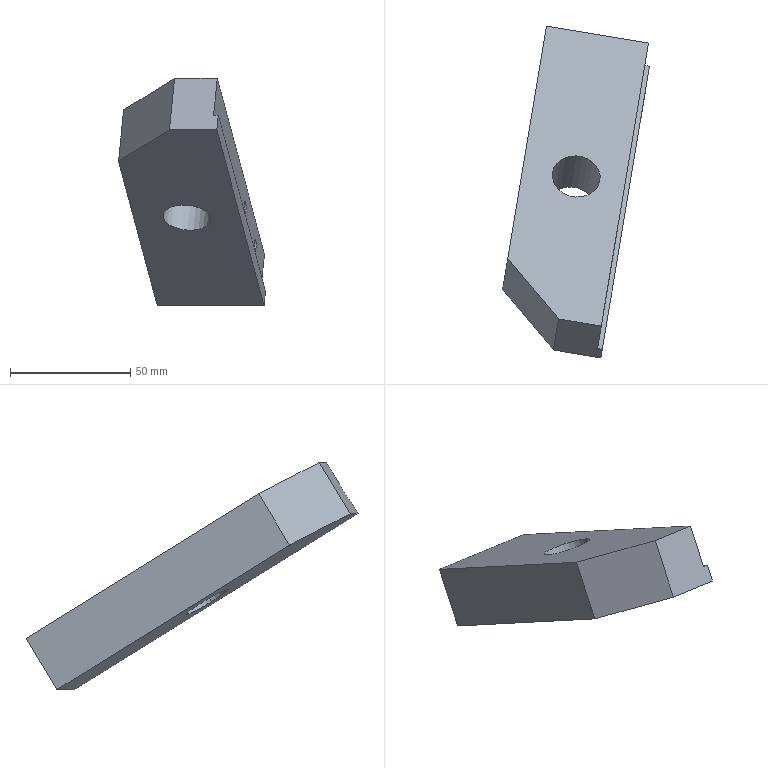Component | SolidWorks | 14AC-24-1-006-1 | 1 solid | 35 faces | box 61.1 x 138.05 x 94.42 mm | volume 135396 mm3 | cylinder 14 | cone 12 | plane 9 | commonest cylinder face diameters 4.2 x8 5 x4 20 x2
build123d program:
from build123d import *

# Parameters (mm, degrees)
SKETCH1_W             = 45
SKETCH1_H             = 140
BOSS_EXTRUDE1_DEPTH   = 25
CUT_EXTRUDE2_DEPTH    = 2
CHAMFER2_SIZE         = 25
M6_TAPPED_HOLE1_D     = 5
M6_TAPPED_HOLE1_DEPTH = 17
M6_TAPPED_HOLE1_TIP   = 1.502
M5_TAPPED_HOLE2_D     = 4.2
M5_TAPPED_HOLE2_DEPTH = 12.4
M5_TAPPED_HOLE2_TIP   = 1.262
SKETCH8_R             = 10
CUT_EXTRUDE3_DEPTH    = 78.661


with BuildPart() as part:
    # Sketch1 → Boss-Extrude1 (new body)
    with BuildSketch(Plane.XY):
        Rectangle(SKETCH1_W, SKETCH1_H)
    extrude(amount=BOSS_EXTRUDE1_DEPTH)

    # Sketch4 → Cut-Extrude2 (cut)
    with BuildSketch(Plane(origin=(22.5, 0, 0), x_dir=(0, 0, -1), z_dir=(1, 0, 0))):
        with BuildLine():
            Line((-18, 70), (0, 70))
            Line((0, 70), (0, -78.5))
            ThreePointArc((0, -78.5), (1.061, -81.061), (-1.5, -80))
            Line((-1.5, -80), (-16.5, -80))
            ThreePointArc((-16.5, -80), (-19.061, -81.061), (-18, -78.5))
            Line((-18, -78.5), (-18, 70))
        make_face()
    extrude(amount=-CUT_EXTRUDE2_DEPTH, mode=Mode.SUBTRACT)

    # Chamfer2
    chamfer2_edges = [part.edges().sort_by_distance(p)[0] for p in [
        (-22.5, 70, 12.5),
    ]]
    chamfer(chamfer2_edges, length=CHAMFER2_SIZE)

    # M6 Tapped Hole1
    with Locations(Plane(origin=(20.5, -48, 9), x_dir=(0, 1, 0), z_dir=(1, 0, 0))):
        with Locations((0, 0), (30, 0)):
            Hole(M6_TAPPED_HOLE1_D / 2, depth=M6_TAPPED_HOLE1_DEPTH)
            with Locations((0, 0, -(M6_TAPPED_HOLE1_DEPTH + M6_TAPPED_HOLE1_TIP / 2))):  # 118° drill point
                Cone(0, M6_TAPPED_HOLE1_D / 2, M6_TAPPED_HOLE1_TIP, mode=Mode.SUBTRACT)

    # M5 Tapped Hole2
    with Locations(Plane(origin=(0, -70, 0), x_dir=(-1, 0, 0), z_dir=(0, -1, 0))):
        with Locations((-12, -4.5), (14, -4.5), (14, -20.5), (-12, -20.5)):
            Hole(M5_TAPPED_HOLE2_D / 2, depth=M5_TAPPED_HOLE2_DEPTH)
            with Locations((0, 0, -(M5_TAPPED_HOLE2_DEPTH + M5_TAPPED_HOLE2_TIP / 2))):  # 118° drill point
                Cone(0, M5_TAPPED_HOLE2_D / 2, M5_TAPPED_HOLE2_TIP, mode=Mode.SUBTRACT)

    # Sketch8 → Cut-Extrude3 (cut, through all)
    with BuildSketch(Plane.XY.offset(25)):
        Circle(SKETCH8_R)
    extrude(amount=-CUT_EXTRUDE3_DEPTH, mode=Mode.SUBTRACT)


solid = part.part

# Placed as in the assembly
solid = solid.moved(Location((401.932, -204.897, -116.607), (148.871, -4.92, 8.082)))
STEP:
#1=COLOUR_RGB('',0.7922,0.8196,0.9333);
#2=FILL_AREA_STYLE_COLOUR('',#1);
#3=FILL_AREA_STYLE('',(#2));
#4=SURFACE_STYLE_FILL_AREA(#3);
#5=SURFACE_SIDE_STYLE('',(#4));
#6=SURFACE_STYLE_USAGE(.BOTH.,#5);
#7=PRESENTATION_STYLE_ASSIGNMENT((#6));
#8=CARTESIAN_POINT('',(15.436,-8.002,-4.591));
#9=VERTEX_POINT('',#8);
#10=CARTESIAN_POINT('',(16.212,-8.131,-4.591));
#11=VERTEX_POINT('',#10);
#12=CARTESIAN_POINT('',(15.824,-8.067,-4.591));
#13=DIRECTION('',(-0.08576,-0.5151,-0.8529));
#14=DIRECTION('',(0.9864,-0.1642,-0.));
#15=AXIS2_PLACEMENT_3D('',#12,#13,#14);
#16=CIRCLE('',#15,0.3937);
#17=EDGE_CURVE('',#9,#11,#16,.T.);
#18=ORIENTED_EDGE('',*,*,#17,.F.);
#19=CARTESIAN_POINT('',(15.351,-8.509,-5.43));
#20=VERTEX_POINT('',#19);
#21=CARTESIAN_POINT('',(15.436,-8.002,-4.591));
#22=DIRECTION('',(-0.08576,-0.5151,-0.8529));
#23=VECTOR('',#22,39.37);
#24=LINE('',#21,#23);
#25=EDGE_CURVE('',#9,#20,#24,.T.);
#26=ORIENTED_EDGE('',*,*,#25,.T.);
#27=CARTESIAN_POINT('',(16.128,-8.638,-5.43));
#28=VERTEX_POINT('',#27);
#29=CARTESIAN_POINT('',(15.74,-8.574,-5.43));
#30=DIRECTION('',(-0.08576,-0.5151,-0.8529));
#31=DIRECTION('',(0.9864,-0.1642,0.));
#32=AXIS2_PLACEMENT_3D('',#29,#30,#31);
#33=CIRCLE('',#32,0.3937);
#34=EDGE_CURVE('',#20,#28,#33,.T.);
#35=ORIENTED_EDGE('',*,*,#34,.T.);
#36=CARTESIAN_POINT('',(16.212,-8.131,-4.591));
#37=DIRECTION('',(-0.08576,-0.5151,-0.8529));
#38=VECTOR('',#37,39.37);
#39=LINE('',#36,#38);
#40=EDGE_CURVE('',#11,#28,#39,.T.);
#41=ORIENTED_EDGE('',*,*,#40,.F.);
#42=EDGE_LOOP('',(#18,#26,#35,#41));
#43=FACE_OUTER_BOUND('',#42,.T.);
#44=CARTESIAN_POINT('',(15.824,-8.067,-4.591));
#45=DIRECTION('',(-0.08576,-0.5151,-0.8529));
#46=DIRECTION('',(0.9864,-0.1642,-0.));
#47=AXIS2_PLACEMENT_3D('',#44,#45,#46);
#48=CYLINDRICAL_SURFACE('',#47,0.3937);
#49=ADVANCED_FACE('',(#43),#48,.F.);
#50=CARTESIAN_POINT('',(16.586,-6.37,-5.997));
#51=VERTEX_POINT('',#50);
#52=CARTESIAN_POINT('',(16.6,-6.285,-5.855));
#53=VERTEX_POINT('',#52);
#54=CARTESIAN_POINT('',(16.593,-6.328,-5.926));
#55=DIRECTION('',(0.1401,0.8413,-0.5222));
#56=DIRECTION('',(0.08576,0.5151,0.8529));
#57=AXIS2_PLACEMENT_3D('',#54,#55,#56);
#58=CIRCLE('',#57,0.08268);
#59=EDGE_CURVE('',#51,#53,#58,.T.);
#60=ORIENTED_EDGE('',*,*,#59,.F.);
#61=CARTESIAN_POINT('',(16.654,-5.96,-6.251));
#62=VERTEX_POINT('',#61);
#63=CARTESIAN_POINT('',(16.654,-5.96,-6.251));
#64=DIRECTION('',(0.1401,0.8413,-0.5222));
#65=VECTOR('',#64,39.37);
#66=LINE('',#63,#65);
#67=EDGE_CURVE('',#51,#62,#66,.T.);
#68=ORIENTED_EDGE('',*,*,#67,.T.);
#69=CARTESIAN_POINT('',(16.668,-5.875,-6.11));
#70=VERTEX_POINT('',#69);
#71=CARTESIAN_POINT('',(16.661,-5.917,-6.181));
#72=DIRECTION('',(0.1401,0.8413,-0.5222));
#73=DIRECTION('',(0.08576,0.5151,0.8529));
#74=AXIS2_PLACEMENT_3D('',#71,#72,#73);
#75=CIRCLE('',#74,0.08268);
#76=EDGE_CURVE('',#62,#70,#75,.T.);
#77=ORIENTED_EDGE('',*,*,#76,.T.);
#78=CARTESIAN_POINT('',(16.668,-5.875,-6.11));
#79=DIRECTION('',(0.1401,0.8413,-0.5222));
#80=VECTOR('',#79,39.37);
#81=LINE('',#78,#80);
#82=EDGE_CURVE('',#53,#70,#81,.T.);
#83=ORIENTED_EDGE('',*,*,#82,.F.);
#84=EDGE_LOOP('',(#60,#68,#77,#83));
#85=FACE_OUTER_BOUND('',#84,.T.);
#86=CARTESIAN_POINT('',(16.661,-5.917,-6.181));
#87=DIRECTION('',(0.1401,0.8413,-0.5222));
#88=DIRECTION('',(0.08576,0.5151,0.8529));
#89=AXIS2_PLACEMENT_3D('',#86,#87,#88);
#90=CYLINDRICAL_SURFACE('',#89,0.08268);
#91=ADVANCED_FACE('',(#85),#90,.F.);
#92=CARTESIAN_POINT('',(16.586,-6.37,-5.9));
#93=VERTEX_POINT('',#92);
#94=CARTESIAN_POINT('',(16.6,-6.285,-5.855));
#95=DIRECTION('',(0.1457,0.8748,0.4621));
#96=VECTOR('',#95,39.37);
#97=LINE('',#94,#96);
#98=EDGE_CURVE('',#93,#53,#97,.T.);
#99=ORIENTED_EDGE('',*,*,#98,.F.);
#100=CARTESIAN_POINT('',(16.586,-6.37,-5.997));
#101=DIRECTION('',(-0.001367,-0.008211,-1.));
#102=VECTOR('',#101,39.37);
#103=LINE('',#100,#102);
#104=EDGE_CURVE('',#93,#51,#103,.T.);
#105=ORIENTED_EDGE('',*,*,#104,.T.);
#106=ORIENTED_EDGE('',*,*,#59,.T.);
#107=EDGE_LOOP('',(#99,#105,#106));
#108=FACE_OUTER_BOUND('',#107,.T.);
#109=CARTESIAN_POINT('',(16.593,-6.328,-5.926));
#110=DIRECTION('',(0.1401,0.8413,-0.5222));
#111=DIRECTION('',(0.08576,0.5151,0.8529));
#112=AXIS2_PLACEMENT_3D('',#109,#110,#111);
#113=CONICAL_SURFACE('',#112,0.08268,1.03);
#114=ADVANCED_FACE('',(#108),#113,.F.);
#115=CARTESIAN_POINT('',(15.576,-6.202,-5.997));
#116=VERTEX_POINT('',#115);
#117=CARTESIAN_POINT('',(15.59,-6.117,-5.855));
#118=VERTEX_POINT('',#117);
#119=CARTESIAN_POINT('',(15.583,-6.16,-5.926));
#120=DIRECTION('',(0.1401,0.8413,-0.5222));
#121=DIRECTION('',(0.08576,0.5151,0.8529));
#122=AXIS2_PLACEMENT_3D('',#119,#120,#121);
#123=CIRCLE('',#122,0.08268);
#124=EDGE_CURVE('',#116,#118,#123,.T.);
#125=ORIENTED_EDGE('',*,*,#124,.F.);
#126=CARTESIAN_POINT('',(15.644,-5.792,-6.251));
#127=VERTEX_POINT('',#126);
#128=CARTESIAN_POINT('',(15.644,-5.792,-6.251));
#129=DIRECTION('',(0.1401,0.8413,-0.5222));
#130=VECTOR('',#129,39.37);
#131=LINE('',#128,#130);
#132=EDGE_CURVE('',#116,#127,#131,.T.);
#133=ORIENTED_EDGE('',*,*,#132,.T.);
#134=CARTESIAN_POINT('',(15.658,-5.707,-6.11));
#135=VERTEX_POINT('',#134);
#136=CARTESIAN_POINT('',(15.651,-5.749,-6.181));
#137=DIRECTION('',(0.1401,0.8413,-0.5222));
#138=DIRECTION('',(0.08576,0.5151,0.8529));
#139=AXIS2_PLACEMENT_3D('',#136,#137,#138);
#140=CIRCLE('',#139,0.08268);
#141=EDGE_CURVE('',#127,#135,#140,.T.);
#142=ORIENTED_EDGE('',*,*,#141,.T.);
#143=CARTESIAN_POINT('',(15.658,-5.707,-6.11));
#144=DIRECTION('',(0.1401,0.8413,-0.5222));
#145=VECTOR('',#144,39.37);
#146=LINE('',#143,#145);
#147=EDGE_CURVE('',#118,#135,#146,.T.);
#148=ORIENTED_EDGE('',*,*,#147,.F.);
#149=EDGE_LOOP('',(#125,#133,#142,#148));
#150=FACE_OUTER_BOUND('',#149,.T.);
#151=CARTESIAN_POINT('',(15.651,-5.749,-6.181));
#152=DIRECTION('',(0.1401,0.8413,-0.5222));
#153=DIRECTION('',(0.08576,0.5151,0.8529));
#154=AXIS2_PLACEMENT_3D('',#151,#152,#153);
#155=CYLINDRICAL_SURFACE('',#154,0.08268);
#156=ADVANCED_FACE('',(#150),#155,.F.);
#157=CARTESIAN_POINT('',(15.576,-6.202,-5.9));
#158=VERTEX_POINT('',#157);
#159=CARTESIAN_POINT('',(15.59,-6.117,-5.855));
#160=DIRECTION('',(0.1457,0.8748,0.4621));
#161=VECTOR('',#160,39.37);
#162=LINE('',#159,#161);
#163=EDGE_CURVE('',#158,#118,#162,.T.);
#164=ORIENTED_EDGE('',*,*,#163,.F.);
#165=CARTESIAN_POINT('',(15.576,-6.202,-5.997));
#166=DIRECTION('',(-0.001367,-0.008211,-1.));
#167=VECTOR('',#166,39.37);
#168=LINE('',#165,#167);
#169=EDGE_CURVE('',#158,#116,#168,.T.);
#170=ORIENTED_EDGE('',*,*,#169,.T.);
#171=ORIENTED_EDGE('',*,*,#124,.T.);
#172=EDGE_LOOP('',(#164,#170,#171));
#173=FACE_OUTER_BOUND('',#172,.T.);
#174=CARTESIAN_POINT('',(15.583,-6.16,-5.926));
#175=DIRECTION('',(0.1401,0.8413,-0.5222));
#176=DIRECTION('',(0.08576,0.5151,0.8529));
#177=AXIS2_PLACEMENT_3D('',#174,#175,#176);
#178=CONICAL_SURFACE('',#177,0.08268,1.03);
#179=ADVANCED_FACE('',(#173),#178,.F.);
#180=CARTESIAN_POINT('',(15.522,-6.527,-6.534));
#181=VERTEX_POINT('',#180);
#182=CARTESIAN_POINT('',(15.536,-6.442,-6.393));
#183=VERTEX_POINT('',#182);
#184=CARTESIAN_POINT('',(15.529,-6.484,-6.463));
#185=DIRECTION('',(0.1401,0.8413,-0.5222));
#186=DIRECTION('',(0.08576,0.5151,0.8529));
#187=AXIS2_PLACEMENT_3D('',#184,#185,#186);
#188=CIRCLE('',#187,0.08268);
#189=EDGE_CURVE('',#181,#183,#188,.T.);
#190=ORIENTED_EDGE('',*,*,#189,.F.);
#191=CARTESIAN_POINT('',(15.59,-6.116,-6.789));
#192=VERTEX_POINT('',#191);
#193=CARTESIAN_POINT('',(15.59,-6.116,-6.789));
#194=DIRECTION('',(0.1401,0.8413,-0.5222));
#195=VECTOR('',#194,39.37);
#196=LINE('',#193,#195);
#197=EDGE_CURVE('',#181,#192,#196,.T.);
#198=ORIENTED_EDGE('',*,*,#197,.T.);
#199=CARTESIAN_POINT('',(15.604,-6.031,-6.648));
#200=VERTEX_POINT('',#199);
#201=CARTESIAN_POINT('',(15.597,-6.074,-6.718));
#202=DIRECTION('',(0.1401,0.8413,-0.5222));
#203=DIRECTION('',(0.08576,0.5151,0.8529));
#204=AXIS2_PLACEMENT_3D('',#201,#202,#203);
#205=CIRCLE('',#204,0.08268);
#206=EDGE_CURVE('',#192,#200,#205,.T.);
#207=ORIENTED_EDGE('',*,*,#206,.T.);
#208=CARTESIAN_POINT('',(15.604,-6.031,-6.648));
#209=DIRECTION('',(0.1401,0.8413,-0.5222));
#210=VECTOR('',#209,39.37);
#211=LINE('',#208,#210);
#212=EDGE_CURVE('',#183,#200,#211,.T.);
#213=ORIENTED_EDGE('',*,*,#212,.F.);
#214=EDGE_LOOP('',(#190,#198,#207,#213));
#215=FACE_OUTER_BOUND('',#214,.T.);
#216=CARTESIAN_POINT('',(15.597,-6.074,-6.718));
#217=DIRECTION('',(0.1401,0.8413,-0.5222));
#218=DIRECTION('',(0.08576,0.5151,0.8529));
#219=AXIS2_PLACEMENT_3D('',#216,#217,#218);
#220=CYLINDRICAL_SURFACE('',#219,0.08268);
#221=ADVANCED_FACE('',(#215),#220,.F.);
#222=CARTESIAN_POINT('',(15.522,-6.526,-6.437));
#223=VERTEX_POINT('',#222);
#224=CARTESIAN_POINT('',(15.536,-6.442,-6.393));
#225=DIRECTION('',(0.1457,0.8748,0.4621));
#226=VECTOR('',#225,39.37);
#227=LINE('',#224,#226);
#228=EDGE_CURVE('',#223,#183,#227,.T.);
#229=ORIENTED_EDGE('',*,*,#228,.F.);
#230=CARTESIAN_POINT('',(15.522,-6.527,-6.534));
#231=DIRECTION('',(-0.001367,-0.008211,-1.));
#232=VECTOR('',#231,39.37);
#233=LINE('',#230,#232);
#234=EDGE_CURVE('',#223,#181,#233,.T.);
#235=ORIENTED_EDGE('',*,*,#234,.T.);
#236=ORIENTED_EDGE('',*,*,#189,.T.);
#237=EDGE_LOOP('',(#229,#235,#236));
#238=FACE_OUTER_BOUND('',#237,.T.);
#239=CARTESIAN_POINT('',(15.529,-6.484,-6.463));
#240=DIRECTION('',(0.1401,0.8413,-0.5222));
#241=DIRECTION('',(0.08576,0.5151,0.8529));
#242=AXIS2_PLACEMENT_3D('',#239,#240,#241);
#243=CONICAL_SURFACE('',#242,0.08268,1.03);
#244=ADVANCED_FACE('',(#238),#243,.F.);
#245=CARTESIAN_POINT('',(16.531,-6.695,-6.534));
#246=VERTEX_POINT('',#245);
#247=CARTESIAN_POINT('',(16.546,-6.61,-6.393));
#248=VERTEX_POINT('',#247);
#249=CARTESIAN_POINT('',(16.539,-6.652,-6.463));
#250=DIRECTION('',(0.1401,0.8413,-0.5222));
#251=DIRECTION('',(0.08576,0.5151,0.8529));
#252=AXIS2_PLACEMENT_3D('',#249,#250,#251);
#253=CIRCLE('',#252,0.08268);
#254=EDGE_CURVE('',#246,#248,#253,.T.);
#255=ORIENTED_EDGE('',*,*,#254,.F.);
#256=CARTESIAN_POINT('',(16.6,-6.284,-6.789));
#257=VERTEX_POINT('',#256);
#258=CARTESIAN_POINT('',(16.6,-6.284,-6.789));
#259=DIRECTION('',(0.1401,0.8413,-0.5222));
#260=VECTOR('',#259,39.37);
#261=LINE('',#258,#260);
#262=EDGE_CURVE('',#246,#257,#261,.T.);
#263=ORIENTED_EDGE('',*,*,#262,.T.);
#264=CARTESIAN_POINT('',(16.614,-6.199,-6.648));
#265=VERTEX_POINT('',#264);
#266=CARTESIAN_POINT('',(16.607,-6.242,-6.718));
#267=DIRECTION('',(0.1401,0.8413,-0.5222));
#268=DIRECTION('',(0.08576,0.5151,0.8529));
#269=AXIS2_PLACEMENT_3D('',#266,#267,#268);
#270=CIRCLE('',#269,0.08268);
#271=EDGE_CURVE('',#257,#265,#270,.T.);
#272=ORIENTED_EDGE('',*,*,#271,.T.);
#273=CARTESIAN_POINT('',(16.614,-6.199,-6.648));
#274=DIRECTION('',(0.1401,0.8413,-0.5222));
#275=VECTOR('',#274,39.37);
#276=LINE('',#273,#275);
#277=EDGE_CURVE('',#248,#265,#276,.T.);
#278=ORIENTED_EDGE('',*,*,#277,.F.);
#279=EDGE_LOOP('',(#255,#263,#272,#278));
#280=FACE_OUTER_BOUND('',#279,.T.);
#281=CARTESIAN_POINT('',(16.607,-6.242,-6.718));
#282=DIRECTION('',(0.1401,0.8413,-0.5222));
#283=DIRECTION('',(0.08576,0.5151,0.8529));
#284=AXIS2_PLACEMENT_3D('',#281,#282,#283);
#285=CYLINDRICAL_SURFACE('',#284,0.08268);
#286=ADVANCED_FACE('',(#280),#285,.F.);
#287=CARTESIAN_POINT('',(16.532,-6.694,-6.437));
#288=VERTEX_POINT('',#287);
#289=CARTESIAN_POINT('',(16.546,-6.61,-6.393));
#290=DIRECTION('',(0.1457,0.8748,0.4621));
#291=VECTOR('',#290,39.37);
#292=LINE('',#289,#291);
#293=EDGE_CURVE('',#288,#248,#292,.T.);
#294=ORIENTED_EDGE('',*,*,#293,.F.);
#295=CARTESIAN_POINT('',(16.531,-6.695,-6.534));
#296=DIRECTION('',(-0.001367,-0.008211,-1.));
#297=VECTOR('',#296,39.37);
#298=LINE('',#295,#297);
#299=EDGE_CURVE('',#288,#246,#298,.T.);
#300=ORIENTED_EDGE('',*,*,#299,.T.);
#301=ORIENTED_EDGE('',*,*,#254,.T.);
#302=EDGE_LOOP('',(#294,#300,#301));
#303=FACE_OUTER_BOUND('',#302,.T.);
#304=CARTESIAN_POINT('',(16.539,-6.652,-6.463));
#305=DIRECTION('',(0.1401,0.8413,-0.5222));
#306=DIRECTION('',(0.08576,0.5151,0.8529));
#307=AXIS2_PLACEMENT_3D('',#304,#305,#306);
#308=CONICAL_SURFACE('',#307,0.08268,1.03);
#309=ADVANCED_FACE('',(#303),#308,.F.);
#310=CARTESIAN_POINT('',(16.186,-6.733,-5.964));
#311=VERTEX_POINT('',#310);
#312=CARTESIAN_POINT('',(16.203,-6.631,-5.796));
#313=VERTEX_POINT('',#312);
#314=CARTESIAN_POINT('',(16.194,-6.682,-5.88));
#315=DIRECTION('',(0.9864,-0.1642,-0.));
#316=DIRECTION('',(0.08576,0.5151,0.8529));
#317=AXIS2_PLACEMENT_3D('',#314,#315,#316);
#318=CIRCLE('',#317,0.09843);
#319=EDGE_CURVE('',#311,#313,#318,.T.);
#320=ORIENTED_EDGE('',*,*,#319,.F.);
#321=CARTESIAN_POINT('',(16.846,-6.843,-5.964));
#322=VERTEX_POINT('',#321);
#323=CARTESIAN_POINT('',(16.846,-6.843,-5.964));
#324=DIRECTION('',(0.9864,-0.1642,-0.));
#325=VECTOR('',#324,39.37);
#326=LINE('',#323,#325);
#327=EDGE_CURVE('',#311,#322,#326,.T.);
#328=ORIENTED_EDGE('',*,*,#327,.T.);
#329=CARTESIAN_POINT('',(16.863,-6.741,-5.796));
#330=VERTEX_POINT('',#329);
#331=CARTESIAN_POINT('',(16.855,-6.792,-5.88));
#332=DIRECTION('',(0.9864,-0.1642,-0.));
#333=DIRECTION('',(0.08576,0.5151,0.8529));
#334=AXIS2_PLACEMENT_3D('',#331,#332,#333);
#335=CIRCLE('',#334,0.09843);
#336=EDGE_CURVE('',#322,#330,#335,.T.);
#337=ORIENTED_EDGE('',*,*,#336,.T.);
#338=CARTESIAN_POINT('',(16.863,-6.741,-5.796));
#339=DIRECTION('',(0.9864,-0.1642,-0.));
#340=VECTOR('',#339,39.37);
#341=LINE('',#338,#340);
#342=EDGE_CURVE('',#313,#330,#341,.T.);
#343=ORIENTED_EDGE('',*,*,#342,.F.);
#344=EDGE_LOOP('',(#320,#328,#337,#343));
#345=FACE_OUTER_BOUND('',#344,.T.);
#346=CARTESIAN_POINT('',(16.855,-6.792,-5.88));
#347=DIRECTION('',(0.9864,-0.1642,-0.));
#348=DIRECTION('',(0.08576,0.5151,0.8529));
#349=AXIS2_PLACEMENT_3D('',#346,#347,#348);
#350=CYLINDRICAL_SURFACE('',#349,0.09843);
#351=ADVANCED_FACE('',(#345),#350,.F.);
#352=CARTESIAN_POINT('',(16.136,-6.672,-5.88));
#353=VERTEX_POINT('',#352);
#354=CARTESIAN_POINT('',(16.203,-6.631,-5.796));
#355=DIRECTION('',(0.5816,0.3569,0.731));
#356=VECTOR('',#355,39.37);
#357=LINE('',#354,#356);
#358=EDGE_CURVE('',#353,#313,#357,.T.);
#359=ORIENTED_EDGE('',*,*,#358,.F.);
#360=CARTESIAN_POINT('',(16.186,-6.733,-5.964));
#361=DIRECTION('',(0.4345,-0.5261,-0.731));
#362=VECTOR('',#361,39.37);
#363=LINE('',#360,#362);
#364=EDGE_CURVE('',#353,#311,#363,.T.);
#365=ORIENTED_EDGE('',*,*,#364,.T.);
#366=ORIENTED_EDGE('',*,*,#319,.T.);
#367=EDGE_LOOP('',(#359,#365,#366));
#368=FACE_OUTER_BOUND('',#367,.T.);
#369=CARTESIAN_POINT('',(16.194,-6.682,-5.88));
#370=DIRECTION('',(0.9864,-0.1642,-0.));
#371=DIRECTION('',(0.08576,0.5151,0.8529));
#372=AXIS2_PLACEMENT_3D('',#369,#370,#371);
#373=CONICAL_SURFACE('',#372,0.09843,1.03);
#374=ADVANCED_FACE('',(#368),#373,.F.);
#375=CARTESIAN_POINT('',(16.02,-7.726,-5.347));
#376=VERTEX_POINT('',#375);
#377=CARTESIAN_POINT('',(16.037,-7.625,-5.179));
#378=VERTEX_POINT('',#377);
#379=CARTESIAN_POINT('',(16.029,-7.676,-5.263));
#380=DIRECTION('',(0.9864,-0.1642,-0.));
#381=DIRECTION('',(0.08576,0.5151,0.8529));
#382=AXIS2_PLACEMENT_3D('',#379,#380,#381);
#383=CIRCLE('',#382,0.09843);
#384=EDGE_CURVE('',#376,#378,#383,.T.);
#385=ORIENTED_EDGE('',*,*,#384,.F.);
#386=CARTESIAN_POINT('',(16.681,-7.836,-5.347));
#387=VERTEX_POINT('',#386);
#388=CARTESIAN_POINT('',(16.681,-7.836,-5.347));
#389=DIRECTION('',(0.9864,-0.1642,-0.));
#390=VECTOR('',#389,39.37);
#391=LINE('',#388,#390);
#392=EDGE_CURVE('',#376,#387,#391,.T.);
#393=ORIENTED_EDGE('',*,*,#392,.T.);
#394=CARTESIAN_POINT('',(16.698,-7.735,-5.179));
#395=VERTEX_POINT('',#394);
#396=CARTESIAN_POINT('',(16.689,-7.786,-5.263));
#397=DIRECTION('',(0.9864,-0.1642,-0.));
#398=DIRECTION('',(0.08576,0.5151,0.8529));
#399=AXIS2_PLACEMENT_3D('',#396,#397,#398);
#400=CIRCLE('',#399,0.09843);
#401=EDGE_CURVE('',#387,#395,#400,.T.);
#402=ORIENTED_EDGE('',*,*,#401,.T.);
#403=CARTESIAN_POINT('',(16.698,-7.735,-5.179));
#404=DIRECTION('',(0.9864,-0.1642,-0.));
#405=VECTOR('',#404,39.37);
#406=LINE('',#403,#405);
#407=EDGE_CURVE('',#378,#395,#406,.T.);
#408=ORIENTED_EDGE('',*,*,#407,.F.);
#409=EDGE_LOOP('',(#385,#393,#402,#408));
#410=FACE_OUTER_BOUND('',#409,.T.);
#411=CARTESIAN_POINT('',(16.689,-7.786,-5.263));
#412=DIRECTION('',(0.9864,-0.1642,-0.));
#413=DIRECTION('',(0.08576,0.5151,0.8529));
#414=AXIS2_PLACEMENT_3D('',#411,#412,#413);
#415=CYLINDRICAL_SURFACE('',#414,0.09843);
#416=ADVANCED_FACE('',(#410),#415,.F.);
#417=CARTESIAN_POINT('',(15.971,-7.666,-5.263));
#418=VERTEX_POINT('',#417);
#419=CARTESIAN_POINT('',(16.037,-7.625,-5.179));
#420=DIRECTION('',(0.5816,0.3569,0.731));
#421=VECTOR('',#420,39.37);
#422=LINE('',#419,#421);
#423=EDGE_CURVE('',#418,#378,#422,.T.);
#424=ORIENTED_EDGE('',*,*,#423,.F.);
#425=CARTESIAN_POINT('',(16.02,-7.726,-5.347));
#426=DIRECTION('',(0.4345,-0.5261,-0.731));
#427=VECTOR('',#426,39.37);
#428=LINE('',#425,#427);
#429=EDGE_CURVE('',#418,#376,#428,.T.);
#430=ORIENTED_EDGE('',*,*,#429,.T.);
#431=ORIENTED_EDGE('',*,*,#384,.T.);
#432=EDGE_LOOP('',(#424,#430,#431));
#433=FACE_OUTER_BOUND('',#432,.T.);
#434=CARTESIAN_POINT('',(16.029,-7.676,-5.263));
#435=DIRECTION('',(0.9864,-0.1642,-0.));
#436=DIRECTION('',(0.08576,0.5151,0.8529));
#437=AXIS2_PLACEMENT_3D('',#434,#435,#436);
#438=CONICAL_SURFACE('',#437,0.09843,1.03);
#439=ADVANCED_FACE('',(#433),#438,.F.);
#440=CARTESIAN_POINT('',(15.824,-8.067,-4.591));
#441=DIRECTION('',(-0.08576,-0.5151,-0.8529));
#442=DIRECTION('',(0.9864,-0.1642,-0.));
#443=AXIS2_PLACEMENT_3D('',#440,#441,#442);
#444=CIRCLE('',#443,0.3937);
#445=EDGE_CURVE('',#11,#9,#444,.T.);
#446=ORIENTED_EDGE('',*,*,#445,.T.);
#447=ORIENTED_EDGE('',*,*,#17,.T.);
#448=EDGE_LOOP('',(#446,#447));
#449=FACE_BOUND('',#448,.T.);
#450=CARTESIAN_POINT('',(14.702,-9.412,-3.666));
#451=VERTEX_POINT('',#450);
#452=CARTESIAN_POINT('',(15.336,-5.603,-6.03));
#453=VERTEX_POINT('',#452);
#454=CARTESIAN_POINT('',(14.564,-10.24,-3.152));
#455=DIRECTION('',(0.1401,0.8413,-0.5222));
#456=VECTOR('',#455,39.37);
#457=LINE('',#454,#456);
#458=EDGE_CURVE('',#451,#453,#457,.T.);
#459=ORIENTED_EDGE('',*,*,#458,.F.);
#460=CARTESIAN_POINT('',(15.535,-10.401,-3.152));
#461=VERTEX_POINT('',#460);
#462=CARTESIAN_POINT('',(14.702,-9.412,-3.666));
#463=DIRECTION('',(0.5985,-0.711,0.3692));
#464=VECTOR('',#463,39.37);
#465=LINE('',#462,#464);
#466=EDGE_CURVE('',#451,#461,#465,.T.);
#467=ORIENTED_EDGE('',*,*,#466,.T.);
#468=CARTESIAN_POINT('',(16.234,-10.518,-3.152));
#469=VERTEX_POINT('',#468);
#470=CARTESIAN_POINT('',(14.564,-10.24,-3.152));
#471=DIRECTION('',(-0.9864,0.1642,0.));
#472=VECTOR('',#471,39.37);
#473=LINE('',#470,#472);
#474=EDGE_CURVE('',#469,#461,#473,.T.);
#475=ORIENTED_EDGE('',*,*,#474,.F.);
#476=CARTESIAN_POINT('',(17.006,-5.881,-6.03));
#477=VERTEX_POINT('',#476);
#478=CARTESIAN_POINT('',(16.62,-8.199,-4.591));
#479=DIRECTION('',(-0.1401,-0.8413,0.5222));
#480=VECTOR('',#479,39.37);
#481=LINE('',#478,#480);
#482=EDGE_CURVE('',#477,#469,#481,.T.);
#483=ORIENTED_EDGE('',*,*,#482,.F.);
#484=CARTESIAN_POINT('',(15.336,-5.603,-6.03));
#485=DIRECTION('',(0.9864,-0.1642,-0.));
#486=VECTOR('',#485,39.37);
#487=LINE('',#484,#486);
#488=EDGE_CURVE('',#453,#477,#487,.T.);
#489=ORIENTED_EDGE('',*,*,#488,.F.);
#490=EDGE_LOOP('',(#459,#467,#475,#483,#489));
#491=FACE_OUTER_BOUND('',#490,.T.);
#492=CARTESIAN_POINT('',(15.824,-8.067,-4.591));
#493=DIRECTION('',(-0.08576,-0.5151,-0.8529));
#494=DIRECTION('',(0.9864,-0.1642,-0.));
#495=AXIS2_PLACEMENT_3D('',#492,#493,#494);
#496=PLANE('',#495);
#497=ADVANCED_FACE('',(#449,#491),#496,.F.);
#498=CARTESIAN_POINT('',(17.,-6.401,-6.869));
#499=VERTEX_POINT('',#498);
#500=CARTESIAN_POINT('',(17.023,-6.259,-6.634));
#501=VERTEX_POINT('',#500);
#502=CARTESIAN_POINT('',(17.,-6.401,-6.869));
#503=DIRECTION('',(0.08576,0.5151,0.8529));
#504=VECTOR('',#503,39.37);
#505=LINE('',#502,#504);
#506=EDGE_CURVE('',#499,#501,#505,.T.);
#507=ORIENTED_EDGE('',*,*,#506,.T.);
#508=CARTESIAN_POINT('',(16.251,-10.896,-3.756));
#509=VERTEX_POINT('',#508);
#510=CARTESIAN_POINT('',(16.251,-10.896,-3.756));
#511=DIRECTION('',(0.1401,0.8413,-0.5222));
#512=VECTOR('',#511,39.37);
#513=LINE('',#510,#512);
#514=EDGE_CURVE('',#509,#501,#513,.T.);
#515=ORIENTED_EDGE('',*,*,#514,.F.);
#516=CARTESIAN_POINT('',(16.227,-11.038,-3.991));
#517=VERTEX_POINT('',#516);
#518=CARTESIAN_POINT('',(16.227,-11.038,-3.991));
#519=DIRECTION('',(0.08576,0.5151,0.8529));
#520=VECTOR('',#519,39.37);
#521=LINE('',#518,#520);
#522=EDGE_CURVE('',#517,#509,#521,.T.);
#523=ORIENTED_EDGE('',*,*,#522,.F.);
#524=CARTESIAN_POINT('',(16.227,-11.038,-3.991));
#525=DIRECTION('',(-0.1401,-0.8413,0.5222));
#526=VECTOR('',#525,39.37);
#527=LINE('',#524,#526);
#528=EDGE_CURVE('',#499,#517,#527,.T.);
#529=ORIENTED_EDGE('',*,*,#528,.F.);
#530=EDGE_LOOP('',(#507,#515,#523,#529));
#531=FACE_OUTER_BOUND('',#530,.T.);
#532=CARTESIAN_POINT('',(16.227,-11.038,-3.991));
#533=DIRECTION('',(-0.9864,0.1642,0.));
#534=DIRECTION('',(0.1401,0.8413,-0.5222));
#535=AXIS2_PLACEMENT_3D('',#532,#533,#534);
#536=PLANE('',#535);
#537=ADVANCED_FACE('',(#531),#536,.F.);
#538=ORIENTED_EDGE('',*,*,#474,.T.);
#539=CARTESIAN_POINT('',(15.451,-10.908,-3.991));
#540=VERTEX_POINT('',#539);
#541=CARTESIAN_POINT('',(15.451,-10.908,-3.991));
#542=DIRECTION('',(-0.08576,-0.5151,-0.8529));
#543=VECTOR('',#542,39.37);
#544=LINE('',#541,#543);
#545=EDGE_CURVE('',#461,#540,#544,.T.);
#546=ORIENTED_EDGE('',*,*,#545,.T.);
#547=CARTESIAN_POINT('',(14.48,-10.747,-3.991));
#548=DIRECTION('',(-0.9864,0.1642,0.));
#549=VECTOR('',#548,39.37);
#550=LINE('',#547,#549);
#551=EDGE_CURVE('',#517,#540,#550,.T.);
#552=ORIENTED_EDGE('',*,*,#551,.F.);
#553=ORIENTED_EDGE('',*,*,#522,.T.);
#554=CARTESIAN_POINT('',(16.173,-10.883,-3.756));
#555=VERTEX_POINT('',#554);
#556=CARTESIAN_POINT('',(16.173,-10.883,-3.756));
#557=DIRECTION('',(0.9864,-0.1642,-0.));
#558=VECTOR('',#557,39.37);
#559=LINE('',#556,#558);
#560=EDGE_CURVE('',#555,#509,#559,.T.);
#561=ORIENTED_EDGE('',*,*,#560,.F.);
#562=CARTESIAN_POINT('',(16.173,-10.883,-3.756));
#563=DIRECTION('',(-0.08576,-0.5151,-0.8529));
#564=VECTOR('',#563,39.37);
#565=LINE('',#562,#564);
#566=EDGE_CURVE('',#469,#555,#565,.T.);
#567=ORIENTED_EDGE('',*,*,#566,.F.);
#568=EDGE_LOOP('',(#538,#546,#552,#553,#561,#567));
#569=FACE_OUTER_BOUND('',#568,.T.);
#570=CARTESIAN_POINT('',(14.48,-10.747,-3.991));
#571=DIRECTION('',(0.1401,0.8413,-0.5222));
#572=DIRECTION('',(0.08576,0.5151,0.8529));
#573=AXIS2_PLACEMENT_3D('',#570,#571,#572);
#574=PLANE('',#573);
#575=ADVANCED_FACE('',(#569),#574,.F.);
#576=CARTESIAN_POINT('',(14.618,-9.919,-4.505));
#577=VERTEX_POINT('',#576);
#578=CARTESIAN_POINT('',(15.252,-6.11,-6.869));
#579=VERTEX_POINT('',#578);
#580=CARTESIAN_POINT('',(14.48,-10.747,-3.991));
#581=DIRECTION('',(0.1401,0.8413,-0.5222));
#582=VECTOR('',#581,39.37);
#583=LINE('',#580,#582);
#584=EDGE_CURVE('',#577,#579,#583,.T.);
#585=ORIENTED_EDGE('',*,*,#584,.F.);
#586=CARTESIAN_POINT('',(14.618,-9.919,-4.505));
#587=DIRECTION('',(0.08576,0.5151,0.8529));
#588=VECTOR('',#587,39.37);
#589=LINE('',#586,#588);
#590=EDGE_CURVE('',#577,#451,#589,.T.);
#591=ORIENTED_EDGE('',*,*,#590,.T.);
#592=ORIENTED_EDGE('',*,*,#458,.T.);
#593=CARTESIAN_POINT('',(15.252,-6.11,-6.869));
#594=DIRECTION('',(0.08576,0.5151,0.8529));
#595=VECTOR('',#594,39.37);
#596=LINE('',#593,#595);
#597=EDGE_CURVE('',#579,#453,#596,.T.);
#598=ORIENTED_EDGE('',*,*,#597,.F.);
#599=EDGE_LOOP('',(#585,#591,#592,#598));
#600=FACE_OUTER_BOUND('',#599,.T.);
#601=CARTESIAN_POINT('',(14.48,-10.747,-3.991));
#602=DIRECTION('',(0.9864,-0.1642,-0.));
#603=DIRECTION('',(-0.1401,-0.8413,0.5222));
#604=AXIS2_PLACEMENT_3D('',#601,#602,#603);
#605=PLANE('',#604);
#606=ADVANCED_FACE('',(#600),#605,.F.);
#607=CARTESIAN_POINT('',(16.661,-5.917,-6.181));
#608=DIRECTION('',(0.1401,0.8413,-0.5222));
#609=DIRECTION('',(0.08576,0.5151,0.8529));
#610=AXIS2_PLACEMENT_3D('',#607,#608,#609);
#611=CIRCLE('',#610,0.08268);
#612=EDGE_CURVE('',#70,#62,#611,.T.);
#613=ORIENTED_EDGE('',*,*,#612,.F.);
#614=ORIENTED_EDGE('',*,*,#76,.F.);
#615=EDGE_LOOP('',(#613,#614));
#616=FACE_BOUND('',#615,.T.);
#617=CARTESIAN_POINT('',(15.651,-5.749,-6.181));
#618=DIRECTION('',(0.1401,0.8413,-0.5222));
#619=DIRECTION('',(0.08576,0.5151,0.8529));
#620=AXIS2_PLACEMENT_3D('',#617,#618,#619);
#621=CIRCLE('',#620,0.08268);
#622=EDGE_CURVE('',#135,#127,#621,.T.);
#623=ORIENTED_EDGE('',*,*,#622,.F.);
#624=ORIENTED_EDGE('',*,*,#141,.F.);
#625=EDGE_LOOP('',(#623,#624));
#626=FACE_BOUND('',#625,.T.);
#627=CARTESIAN_POINT('',(15.597,-6.074,-6.718));
#628=DIRECTION('',(0.1401,0.8413,-0.5222));
#629=DIRECTION('',(0.08576,0.5151,0.8529));
#630=AXIS2_PLACEMENT_3D('',#627,#628,#629);
#631=CIRCLE('',#630,0.08268);
#632=EDGE_CURVE('',#200,#192,#631,.T.);
#633=ORIENTED_EDGE('',*,*,#632,.F.);
#634=ORIENTED_EDGE('',*,*,#206,.F.);
#635=EDGE_LOOP('',(#633,#634));
#636=FACE_BOUND('',#635,.T.);
#637=CARTESIAN_POINT('',(16.607,-6.242,-6.718));
#638=DIRECTION('',(0.1401,0.8413,-0.5222));
#639=DIRECTION('',(0.08576,0.5151,0.8529));
#640=AXIS2_PLACEMENT_3D('',#637,#638,#639);
#641=CIRCLE('',#640,0.08268);
#642=EDGE_CURVE('',#265,#257,#641,.T.);
#643=ORIENTED_EDGE('',*,*,#642,.F.);
#644=ORIENTED_EDGE('',*,*,#271,.F.);
#645=EDGE_LOOP('',(#643,#644));
#646=FACE_BOUND('',#645,.T.);
#647=CARTESIAN_POINT('',(16.945,-6.246,-6.634));
#648=VERTEX_POINT('',#647);
#649=CARTESIAN_POINT('',(16.922,-6.388,-6.869));
#650=DIRECTION('',(0.08576,0.5151,0.8529));
#651=VECTOR('',#650,39.37);
#652=LINE('',#649,#651);
#653=EDGE_CURVE('',#648,#477,#652,.T.);
#654=ORIENTED_EDGE('',*,*,#653,.F.);
#655=CARTESIAN_POINT('',(15.276,-5.968,-6.634));
#656=DIRECTION('',(0.9864,-0.1642,-0.));
#657=VECTOR('',#656,39.37);
#658=LINE('',#655,#657);
#659=EDGE_CURVE('',#648,#501,#658,.T.);
#660=ORIENTED_EDGE('',*,*,#659,.T.);
#661=ORIENTED_EDGE('',*,*,#506,.F.);
#662=CARTESIAN_POINT('',(15.252,-6.11,-6.869));
#663=DIRECTION('',(0.9864,-0.1642,-0.));
#664=VECTOR('',#663,39.37);
#665=LINE('',#662,#664);
#666=EDGE_CURVE('',#579,#499,#665,.T.);
#667=ORIENTED_EDGE('',*,*,#666,.F.);
#668=ORIENTED_EDGE('',*,*,#597,.T.);
#669=ORIENTED_EDGE('',*,*,#488,.T.);
#670=EDGE_LOOP('',(#654,#660,#661,#667,#668,#669));
#671=FACE_OUTER_BOUND('',#670,.T.);
#672=CARTESIAN_POINT('',(15.252,-6.11,-6.869));
#673=DIRECTION('',(-0.1401,-0.8413,0.5222));
#674=DIRECTION('',(-0.08576,-0.5151,-0.8529));
#675=AXIS2_PLACEMENT_3D('',#672,#673,#674);
#676=PLANE('',#675);
#677=ADVANCED_FACE('',(#616,#626,#636,#646,#671),#676,.F.);
#678=CARTESIAN_POINT('',(15.74,-8.574,-5.43));
#679=DIRECTION('',(-0.08576,-0.5151,-0.8529));
#680=DIRECTION('',(0.9864,-0.1642,0.));
#681=AXIS2_PLACEMENT_3D('',#678,#679,#680);
#682=CIRCLE('',#681,0.3937);
#683=EDGE_CURVE('',#28,#20,#682,.T.);
#684=ORIENTED_EDGE('',*,*,#683,.F.);
#685=ORIENTED_EDGE('',*,*,#34,.F.);
#686=EDGE_LOOP('',(#684,#685));
#687=FACE_BOUND('',#686,.T.);
#688=ORIENTED_EDGE('',*,*,#551,.T.);
#689=CARTESIAN_POINT('',(14.243,-9.473,-4.736));
#690=DIRECTION('',(-0.5985,0.711,-0.3692));
#691=VECTOR('',#690,39.37);
#692=LINE('',#689,#691);
#693=EDGE_CURVE('',#540,#577,#692,.T.);
#694=ORIENTED_EDGE('',*,*,#693,.T.);
#695=ORIENTED_EDGE('',*,*,#584,.T.);
#696=ORIENTED_EDGE('',*,*,#666,.T.);
#697=ORIENTED_EDGE('',*,*,#528,.T.);
#698=EDGE_LOOP('',(#688,#694,#695,#696,#697));
#699=FACE_OUTER_BOUND('',#698,.T.);
#700=CARTESIAN_POINT('',(15.74,-8.574,-5.43));
#701=DIRECTION('',(-0.08576,-0.5151,-0.8529));
#702=DIRECTION('',(0.9864,-0.1642,-0.));
#703=AXIS2_PLACEMENT_3D('',#700,#701,#702);
#704=PLANE('',#703);
#705=ADVANCED_FACE('',(#687,#699),#704,.T.);
#706=CARTESIAN_POINT('',(16.173,-10.883,-3.756));
#707=DIRECTION('',(0.1401,0.8413,-0.5222));
#708=VECTOR('',#707,39.37);
#709=LINE('',#706,#708);
#710=EDGE_CURVE('',#555,#648,#709,.T.);
#711=ORIENTED_EDGE('',*,*,#710,.F.);
#712=ORIENTED_EDGE('',*,*,#560,.T.);
#713=ORIENTED_EDGE('',*,*,#514,.T.);
#714=ORIENTED_EDGE('',*,*,#659,.F.);
#715=EDGE_LOOP('',(#711,#712,#713,#714));
#716=FACE_OUTER_BOUND('',#715,.T.);
#717=CARTESIAN_POINT('',(16.173,-10.883,-3.756));
#718=DIRECTION('',(-0.08576,-0.5151,-0.8529));
#719=DIRECTION('',(0.1401,0.8413,-0.5222));
#720=AXIS2_PLACEMENT_3D('',#717,#718,#719);
#721=PLANE('',#720);
#722=ADVANCED_FACE('',(#716),#721,.F.);
#723=CARTESIAN_POINT('',(16.855,-6.792,-5.88));
#724=DIRECTION('',(0.9864,-0.1642,-0.));
#725=DIRECTION('',(0.08576,0.5151,0.8529));
#726=AXIS2_PLACEMENT_3D('',#723,#724,#725);
#727=CIRCLE('',#726,0.09843);
#728=EDGE_CURVE('',#330,#322,#727,.T.);
#729=ORIENTED_EDGE('',*,*,#728,.F.);
#730=ORIENTED_EDGE('',*,*,#336,.F.);
#731=EDGE_LOOP('',(#729,#730));
#732=FACE_BOUND('',#731,.T.);
#733=CARTESIAN_POINT('',(16.689,-7.786,-5.263));
#734=DIRECTION('',(0.9864,-0.1642,-0.));
#735=DIRECTION('',(0.08576,0.5151,0.8529));
#736=AXIS2_PLACEMENT_3D('',#733,#734,#735);
#737=CIRCLE('',#736,0.09843);
#738=EDGE_CURVE('',#395,#387,#737,.T.);
#739=ORIENTED_EDGE('',*,*,#738,.F.);
#740=ORIENTED_EDGE('',*,*,#401,.F.);
#741=EDGE_LOOP('',(#739,#740));
#742=FACE_BOUND('',#741,.T.);
#743=ORIENTED_EDGE('',*,*,#653,.T.);
#744=ORIENTED_EDGE('',*,*,#482,.T.);
#745=ORIENTED_EDGE('',*,*,#566,.T.);
#746=ORIENTED_EDGE('',*,*,#710,.T.);
#747=EDGE_LOOP('',(#743,#744,#745,#746));
#748=FACE_OUTER_BOUND('',#747,.T.);
#749=CARTESIAN_POINT('',(17.001,-5.915,-6.84));
#750=DIRECTION('',(0.9864,-0.1642,-0.));
#751=DIRECTION('',(-0.1401,-0.8413,0.5222));
#752=AXIS2_PLACEMENT_3D('',#749,#750,#751);
#753=PLANE('',#752);
#754=ADVANCED_FACE('',(#732,#742,#748),#753,.T.);
#755=ORIENTED_EDGE('',*,*,#693,.F.);
#756=ORIENTED_EDGE('',*,*,#545,.F.);
#757=ORIENTED_EDGE('',*,*,#466,.F.);
#758=ORIENTED_EDGE('',*,*,#590,.F.);
#759=EDGE_LOOP('',(#755,#756,#757,#758));
#760=FACE_OUTER_BOUND('',#759,.T.);
#761=CARTESIAN_POINT('',(14.618,-9.919,-4.505));
#762=DIRECTION('',(0.7966,0.4787,-0.3692));
#763=DIRECTION('',(0.08576,0.5151,0.8529));
#764=AXIS2_PLACEMENT_3D('',#761,#762,#763);
#765=PLANE('',#764);
#766=ADVANCED_FACE('',(#760),#765,.F.);
#767=ORIENTED_EDGE('',*,*,#429,.F.);
#768=ORIENTED_EDGE('',*,*,#423,.T.);
#769=CARTESIAN_POINT('',(16.029,-7.676,-5.263));
#770=DIRECTION('',(0.9864,-0.1642,-0.));
#771=DIRECTION('',(0.08576,0.5151,0.8529));
#772=AXIS2_PLACEMENT_3D('',#769,#770,#771);
#773=CIRCLE('',#772,0.09843);
#774=EDGE_CURVE('',#378,#376,#773,.T.);
#775=ORIENTED_EDGE('',*,*,#774,.T.);
#776=EDGE_LOOP('',(#767,#768,#775));
#777=FACE_OUTER_BOUND('',#776,.T.);
#778=CARTESIAN_POINT('',(16.029,-7.676,-5.263));
#779=DIRECTION('',(0.9864,-0.1642,-0.));
#780=DIRECTION('',(0.08576,0.5151,0.8529));
#781=AXIS2_PLACEMENT_3D('',#778,#779,#780);
#782=CONICAL_SURFACE('',#781,0.09843,1.03);
#783=ADVANCED_FACE('',(#777),#782,.F.);
#784=ORIENTED_EDGE('',*,*,#392,.F.);
#785=ORIENTED_EDGE('',*,*,#774,.F.);
#786=ORIENTED_EDGE('',*,*,#407,.T.);
#787=ORIENTED_EDGE('',*,*,#738,.T.);
#788=EDGE_LOOP('',(#784,#785,#786,#787));
#789=FACE_OUTER_BOUND('',#788,.T.);
#790=CARTESIAN_POINT('',(16.689,-7.786,-5.263));
#791=DIRECTION('',(0.9864,-0.1642,-0.));
#792=DIRECTION('',(0.08576,0.5151,0.8529));
#793=AXIS2_PLACEMENT_3D('',#790,#791,#792);
#794=CYLINDRICAL_SURFACE('',#793,0.09843);
#795=ADVANCED_FACE('',(#789),#794,.F.);
#796=ORIENTED_EDGE('',*,*,#364,.F.);
#797=ORIENTED_EDGE('',*,*,#358,.T.);
#798=CARTESIAN_POINT('',(16.194,-6.682,-5.88));
#799=DIRECTION('',(0.9864,-0.1642,-0.));
#800=DIRECTION('',(0.08576,0.5151,0.8529));
#801=AXIS2_PLACEMENT_3D('',#798,#799,#800);
#802=CIRCLE('',#801,0.09843);
#803=EDGE_CURVE('',#313,#311,#802,.T.);
#804=ORIENTED_EDGE('',*,*,#803,.T.);
#805=EDGE_LOOP('',(#796,#797,#804));
#806=FACE_OUTER_BOUND('',#805,.T.);
#807=CARTESIAN_POINT('',(16.194,-6.682,-5.88));
#808=DIRECTION('',(0.9864,-0.1642,-0.));
#809=DIRECTION('',(0.08576,0.5151,0.8529));
#810=AXIS2_PLACEMENT_3D('',#807,#808,#809);
#811=CONICAL_SURFACE('',#810,0.09843,1.03);
#812=ADVANCED_FACE('',(#806),#811,.F.);
#813=ORIENTED_EDGE('',*,*,#327,.F.);
#814=ORIENTED_EDGE('',*,*,#803,.F.);
#815=ORIENTED_EDGE('',*,*,#342,.T.);
#816=ORIENTED_EDGE('',*,*,#728,.T.);
#817=EDGE_LOOP('',(#813,#814,#815,#816));
#818=FACE_OUTER_BOUND('',#817,.T.);
#819=CARTESIAN_POINT('',(16.855,-6.792,-5.88));
#820=DIRECTION('',(0.9864,-0.1642,-0.));
#821=DIRECTION('',(0.08576,0.5151,0.8529));
#822=AXIS2_PLACEMENT_3D('',#819,#820,#821);
#823=CYLINDRICAL_SURFACE('',#822,0.09843);
#824=ADVANCED_FACE('',(#818),#823,.F.);
#825=ORIENTED_EDGE('',*,*,#299,.F.);
#826=ORIENTED_EDGE('',*,*,#293,.T.);
#827=CARTESIAN_POINT('',(16.539,-6.652,-6.463));
#828=DIRECTION('',(0.1401,0.8413,-0.5222));
#829=DIRECTION('',(0.08576,0.5151,0.8529));
#830=AXIS2_PLACEMENT_3D('',#827,#828,#829);
#831=CIRCLE('',#830,0.08268);
#832=EDGE_CURVE('',#248,#246,#831,.T.);
#833=ORIENTED_EDGE('',*,*,#832,.T.);
#834=EDGE_LOOP('',(#825,#826,#833));
#835=FACE_OUTER_BOUND('',#834,.T.);
#836=CARTESIAN_POINT('',(16.539,-6.652,-6.463));
#837=DIRECTION('',(0.1401,0.8413,-0.5222));
#838=DIRECTION('',(0.08576,0.5151,0.8529));
#839=AXIS2_PLACEMENT_3D('',#836,#837,#838);
#840=CONICAL_SURFACE('',#839,0.08268,1.03);
#841=ADVANCED_FACE('',(#835),#840,.F.);
#842=ORIENTED_EDGE('',*,*,#262,.F.);
#843=ORIENTED_EDGE('',*,*,#832,.F.);
#844=ORIENTED_EDGE('',*,*,#277,.T.);
#845=ORIENTED_EDGE('',*,*,#642,.T.);
#846=EDGE_LOOP('',(#842,#843,#844,#845));
#847=FACE_OUTER_BOUND('',#846,.T.);
#848=CARTESIAN_POINT('',(16.607,-6.242,-6.718));
#849=DIRECTION('',(0.1401,0.8413,-0.5222));
#850=DIRECTION('',(0.08576,0.5151,0.8529));
#851=AXIS2_PLACEMENT_3D('',#848,#849,#850);
#852=CYLINDRICAL_SURFACE('',#851,0.08268);
#853=ADVANCED_FACE('',(#847),#852,.F.);
#854=ORIENTED_EDGE('',*,*,#234,.F.);
#855=ORIENTED_EDGE('',*,*,#228,.T.);
#856=CARTESIAN_POINT('',(15.529,-6.484,-6.463));
#857=DIRECTION('',(0.1401,0.8413,-0.5222));
#858=DIRECTION('',(0.08576,0.5151,0.8529));
#859=AXIS2_PLACEMENT_3D('',#856,#857,#858);
#860=CIRCLE('',#859,0.08268);
#861=EDGE_CURVE('',#183,#181,#860,.T.);
#862=ORIENTED_EDGE('',*,*,#861,.T.);
#863=EDGE_LOOP('',(#854,#855,#862));
#864=FACE_OUTER_BOUND('',#863,.T.);
#865=CARTESIAN_POINT('',(15.529,-6.484,-6.463));
#866=DIRECTION('',(0.1401,0.8413,-0.5222));
#867=DIRECTION('',(0.08576,0.5151,0.8529));
#868=AXIS2_PLACEMENT_3D('',#865,#866,#867);
#869=CONICAL_SURFACE('',#868,0.08268,1.03);
#870=ADVANCED_FACE('',(#864),#869,.F.);
#871=ORIENTED_EDGE('',*,*,#197,.F.);
#872=ORIENTED_EDGE('',*,*,#861,.F.);
#873=ORIENTED_EDGE('',*,*,#212,.T.);
#874=ORIENTED_EDGE('',*,*,#632,.T.);
#875=EDGE_LOOP('',(#871,#872,#873,#874));
#876=FACE_OUTER_BOUND('',#875,.T.);
#877=CARTESIAN_POINT('',(15.597,-6.074,-6.718));
#878=DIRECTION('',(0.1401,0.8413,-0.5222));
#879=DIRECTION('',(0.08576,0.5151,0.8529));
#880=AXIS2_PLACEMENT_3D('',#877,#878,#879);
#881=CYLINDRICAL_SURFACE('',#880,0.08268);
#882=ADVANCED_FACE('',(#876),#881,.F.);
#883=ORIENTED_EDGE('',*,*,#169,.F.);
#884=ORIENTED_EDGE('',*,*,#163,.T.);
#885=CARTESIAN_POINT('',(15.583,-6.16,-5.926));
#886=DIRECTION('',(0.1401,0.8413,-0.5222));
#887=DIRECTION('',(0.08576,0.5151,0.8529));
#888=AXIS2_PLACEMENT_3D('',#885,#886,#887);
#889=CIRCLE('',#888,0.08268);
#890=EDGE_CURVE('',#118,#116,#889,.T.);
#891=ORIENTED_EDGE('',*,*,#890,.T.);
#892=EDGE_LOOP('',(#883,#884,#891));
#893=FACE_OUTER_BOUND('',#892,.T.);
#894=CARTESIAN_POINT('',(15.583,-6.16,-5.926));
#895=DIRECTION('',(0.1401,0.8413,-0.5222));
#896=DIRECTION('',(0.08576,0.5151,0.8529));
#897=AXIS2_PLACEMENT_3D('',#894,#895,#896);
#898=CONICAL_SURFACE('',#897,0.08268,1.03);
#899=ADVANCED_FACE('',(#893),#898,.F.);
#900=ORIENTED_EDGE('',*,*,#132,.F.);
#901=ORIENTED_EDGE('',*,*,#890,.F.);
#902=ORIENTED_EDGE('',*,*,#147,.T.);
#903=ORIENTED_EDGE('',*,*,#622,.T.);
#904=EDGE_LOOP('',(#900,#901,#902,#903));
#905=FACE_OUTER_BOUND('',#904,.T.);
#906=CARTESIAN_POINT('',(15.651,-5.749,-6.181));
#907=DIRECTION('',(0.1401,0.8413,-0.5222));
#908=DIRECTION('',(0.08576,0.5151,0.8529));
#909=AXIS2_PLACEMENT_3D('',#906,#907,#908);
#910=CYLINDRICAL_SURFACE('',#909,0.08268);
#911=ADVANCED_FACE('',(#905),#910,.F.);
#912=ORIENTED_EDGE('',*,*,#104,.F.);
#913=ORIENTED_EDGE('',*,*,#98,.T.);
#914=CARTESIAN_POINT('',(16.593,-6.328,-5.926));
#915=DIRECTION('',(0.1401,0.8413,-0.5222));
#916=DIRECTION('',(0.08576,0.5151,0.8529));
#917=AXIS2_PLACEMENT_3D('',#914,#915,#916);
#918=CIRCLE('',#917,0.08268);
#919=EDGE_CURVE('',#53,#51,#918,.T.);
#920=ORIENTED_EDGE('',*,*,#919,.T.);
#921=EDGE_LOOP('',(#912,#913,#920));
#922=FACE_OUTER_BOUND('',#921,.T.);
#923=CARTESIAN_POINT('',(16.593,-6.328,-5.926));
#924=DIRECTION('',(0.1401,0.8413,-0.5222));
#925=DIRECTION('',(0.08576,0.5151,0.8529));
#926=AXIS2_PLACEMENT_3D('',#923,#924,#925);
#927=CONICAL_SURFACE('',#926,0.08268,1.03);
#928=ADVANCED_FACE('',(#922),#927,.F.);
#929=ORIENTED_EDGE('',*,*,#67,.F.);
#930=ORIENTED_EDGE('',*,*,#919,.F.);
#931=ORIENTED_EDGE('',*,*,#82,.T.);
#932=ORIENTED_EDGE('',*,*,#612,.T.);
#933=EDGE_LOOP('',(#929,#930,#931,#932));
#934=FACE_OUTER_BOUND('',#933,.T.);
#935=CARTESIAN_POINT('',(16.661,-5.917,-6.181));
#936=DIRECTION('',(0.1401,0.8413,-0.5222));
#937=DIRECTION('',(0.08576,0.5151,0.8529));
#938=AXIS2_PLACEMENT_3D('',#935,#936,#937);
#939=CYLINDRICAL_SURFACE('',#938,0.08268);
#940=ADVANCED_FACE('',(#934),#939,.F.);
#941=ORIENTED_EDGE('',*,*,#25,.F.);
#942=ORIENTED_EDGE('',*,*,#445,.F.);
#943=ORIENTED_EDGE('',*,*,#40,.T.);
#944=ORIENTED_EDGE('',*,*,#683,.T.);
#945=EDGE_LOOP('',(#941,#942,#943,#944));
#946=FACE_OUTER_BOUND('',#945,.T.);
#947=CARTESIAN_POINT('',(15.824,-8.067,-4.591));
#948=DIRECTION('',(-0.08576,-0.5151,-0.8529));
#949=DIRECTION('',(0.9864,-0.1642,-0.));
#950=AXIS2_PLACEMENT_3D('',#947,#948,#949);
#951=CYLINDRICAL_SURFACE('',#950,0.3937);
#952=ADVANCED_FACE('',(#946),#951,.F.);
#953=CLOSED_SHELL('',(#49,#91,#114,#156,#179,#221,#244,#286,#309,#351,#374,#416,#439,#497,#537,#575,#606,#677,#705,#722,#754,#766,#783,#795,#812,#824,#841,#853,#870,#882,#899,#911,#928,#940,#952));
#954=MANIFOLD_SOLID_BREP('',#953);
#955=STYLED_ITEM('',(#7),#954);
#956=PRESENTATION_LAYER_ASSIGNMENT('','',(#955));
#957=(LENGTH_UNIT()NAMED_UNIT(*)SI_UNIT($,.METRE.));
#958=LENGTH_MEASURE_WITH_UNIT(LENGTH_MEASURE(0.0254),#957);
#959=DIMENSIONAL_EXPONENTS(1.,0.,0.,0.,0.,0.,0.);
#960=(CONVERSION_BASED_UNIT('',#958)LENGTH_UNIT()NAMED_UNIT(#959));
#961=UNCERTAINTY_MEASURE_WITH_UNIT(LENGTH_MEASURE(0.00001),#960,'','');
#962=(NAMED_UNIT(*)PLANE_ANGLE_UNIT()SI_UNIT($,.RADIAN.));
#963=(NAMED_UNIT(*)SI_UNIT($,.STERADIAN.)SOLID_ANGLE_UNIT());
#964=(GEOMETRIC_REPRESENTATION_CONTEXT(3)GLOBAL_UNCERTAINTY_ASSIGNED_CONTEXT((#961))GLOBAL_UNIT_ASSIGNED_CONTEXT((#960,#962,#963))REPRESENTATION_CONTEXT('',''));
#965=MECHANICAL_DESIGN_GEOMETRIC_PRESENTATION_REPRESENTATION('',(#955),#964);
#966=CARTESIAN_POINT('',(0.,0.,0.));
#967=DIRECTION('',(0.,0.,1.));
#968=DIRECTION('',(1.,0.,0.));
#969=AXIS2_PLACEMENT_3D('',#966,#967,#968);
#970=(LENGTH_UNIT()NAMED_UNIT(*)SI_UNIT($,.METRE.));
#971=LENGTH_MEASURE_WITH_UNIT(LENGTH_MEASURE(0.0254),#970);
#972=DIMENSIONAL_EXPONENTS(1.,0.,0.,0.,0.,0.,0.);
#973=(CONVERSION_BASED_UNIT('',#971)LENGTH_UNIT()NAMED_UNIT(#972));
#974=UNCERTAINTY_MEASURE_WITH_UNIT(LENGTH_MEASURE(0.00001),#973,'','');
#975=(NAMED_UNIT(*)PLANE_ANGLE_UNIT()SI_UNIT($,.RADIAN.));
#976=(NAMED_UNIT(*)SI_UNIT($,.STERADIAN.)SOLID_ANGLE_UNIT());
#977=(GEOMETRIC_REPRESENTATION_CONTEXT(3)GLOBAL_UNCERTAINTY_ASSIGNED_CONTEXT((#974))GLOBAL_UNIT_ASSIGNED_CONTEXT((#973,#975,#976))REPRESENTATION_CONTEXT('',''));
#978=ADVANCED_BREP_SHAPE_REPRESENTATION('',(#954,#969),#977);